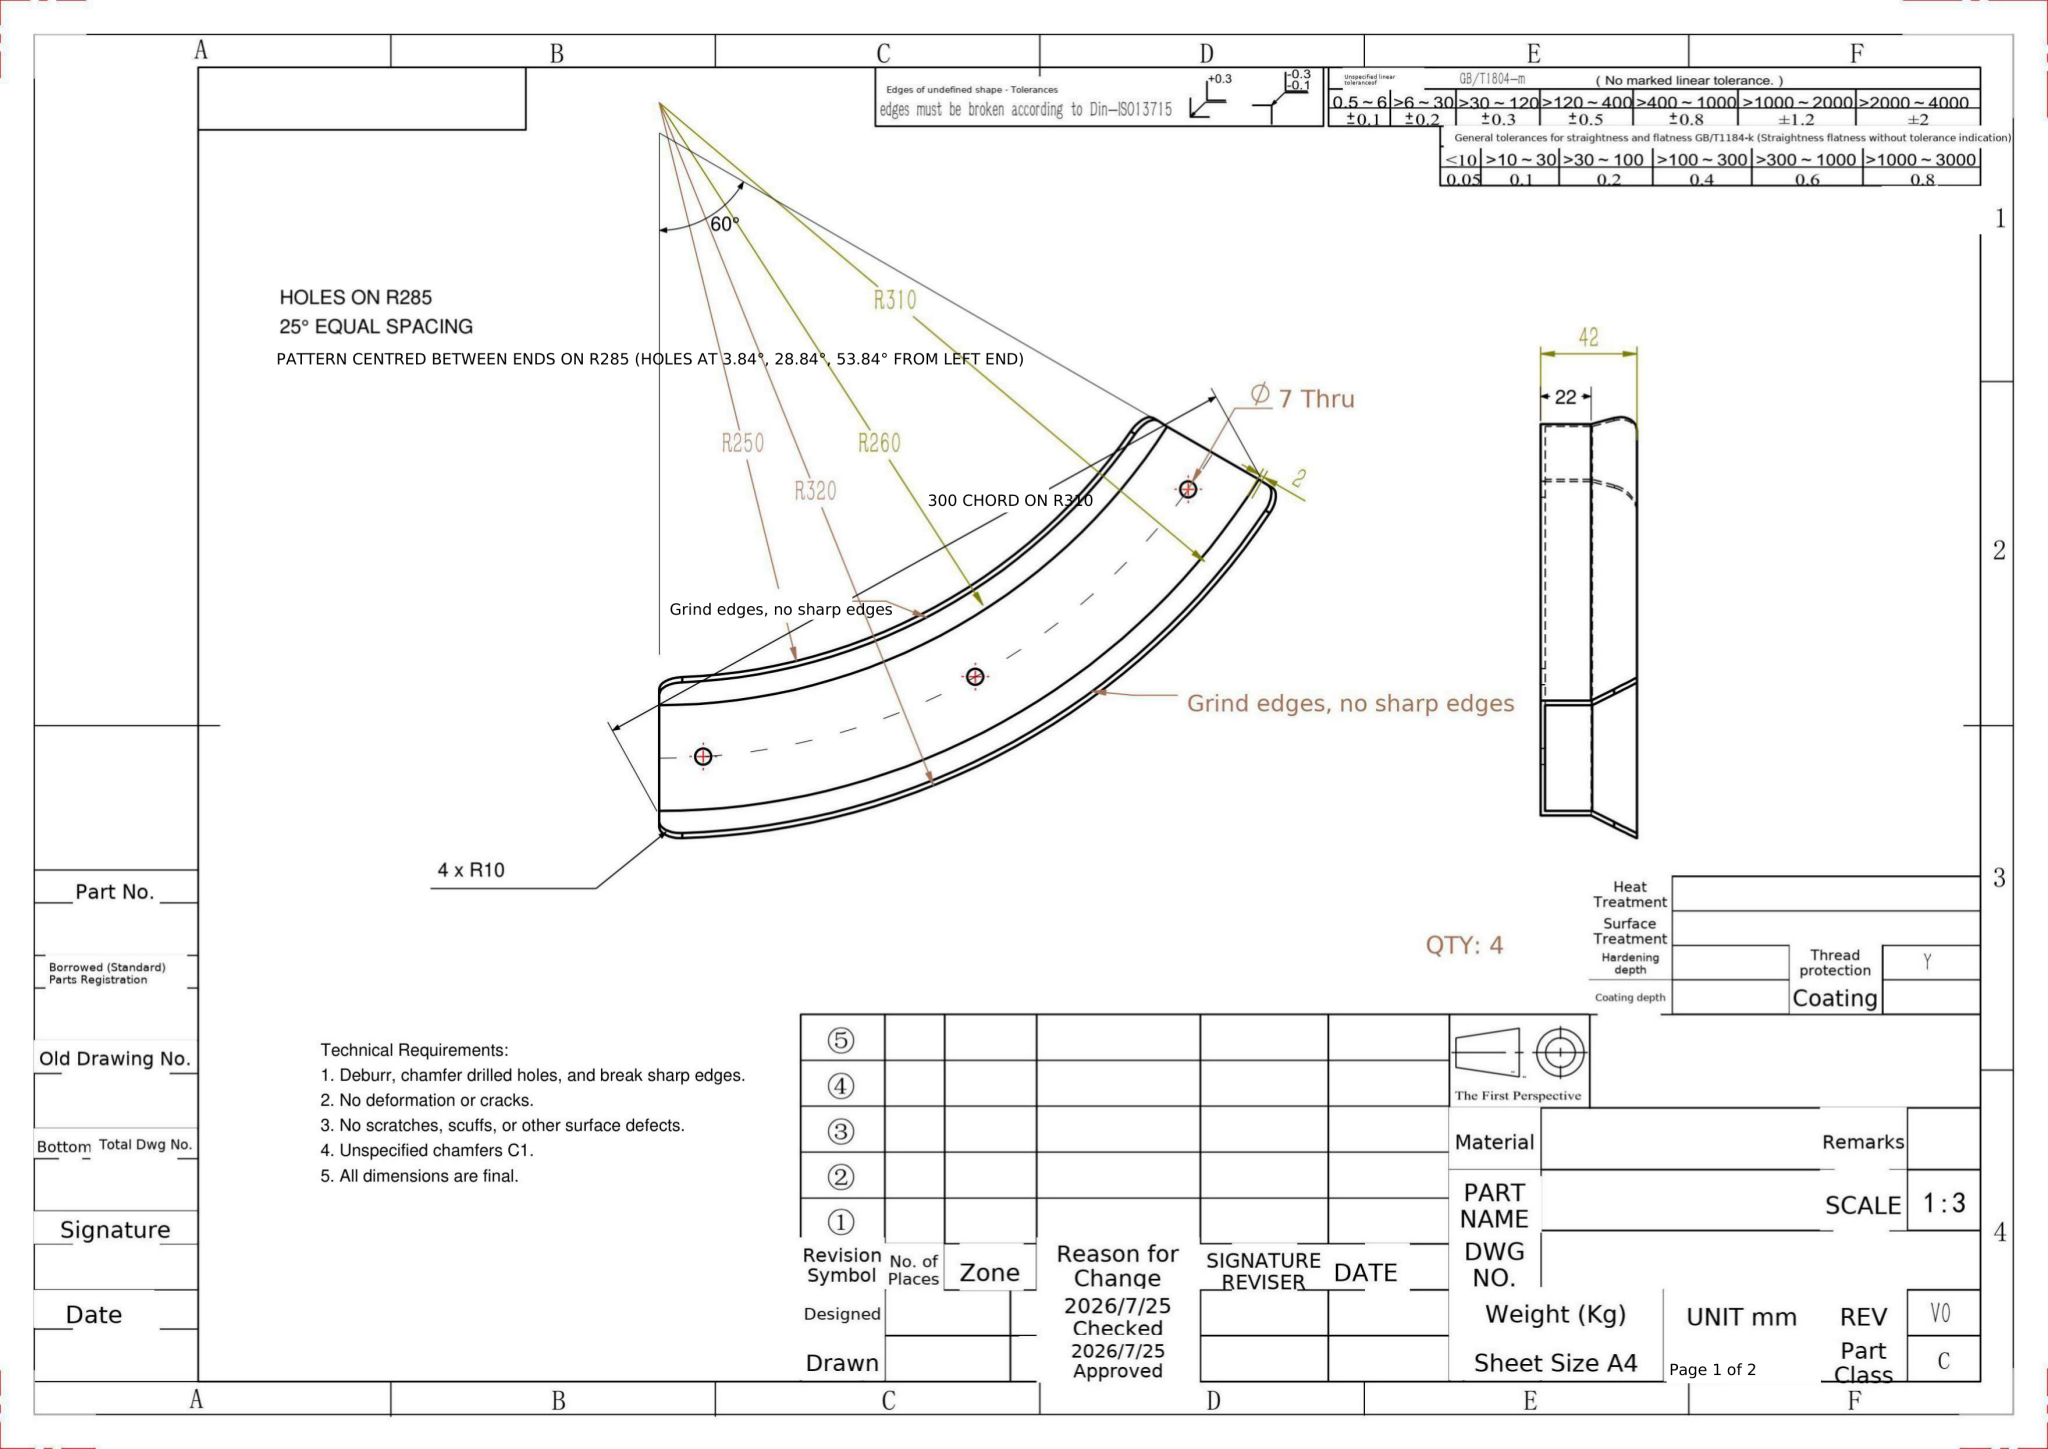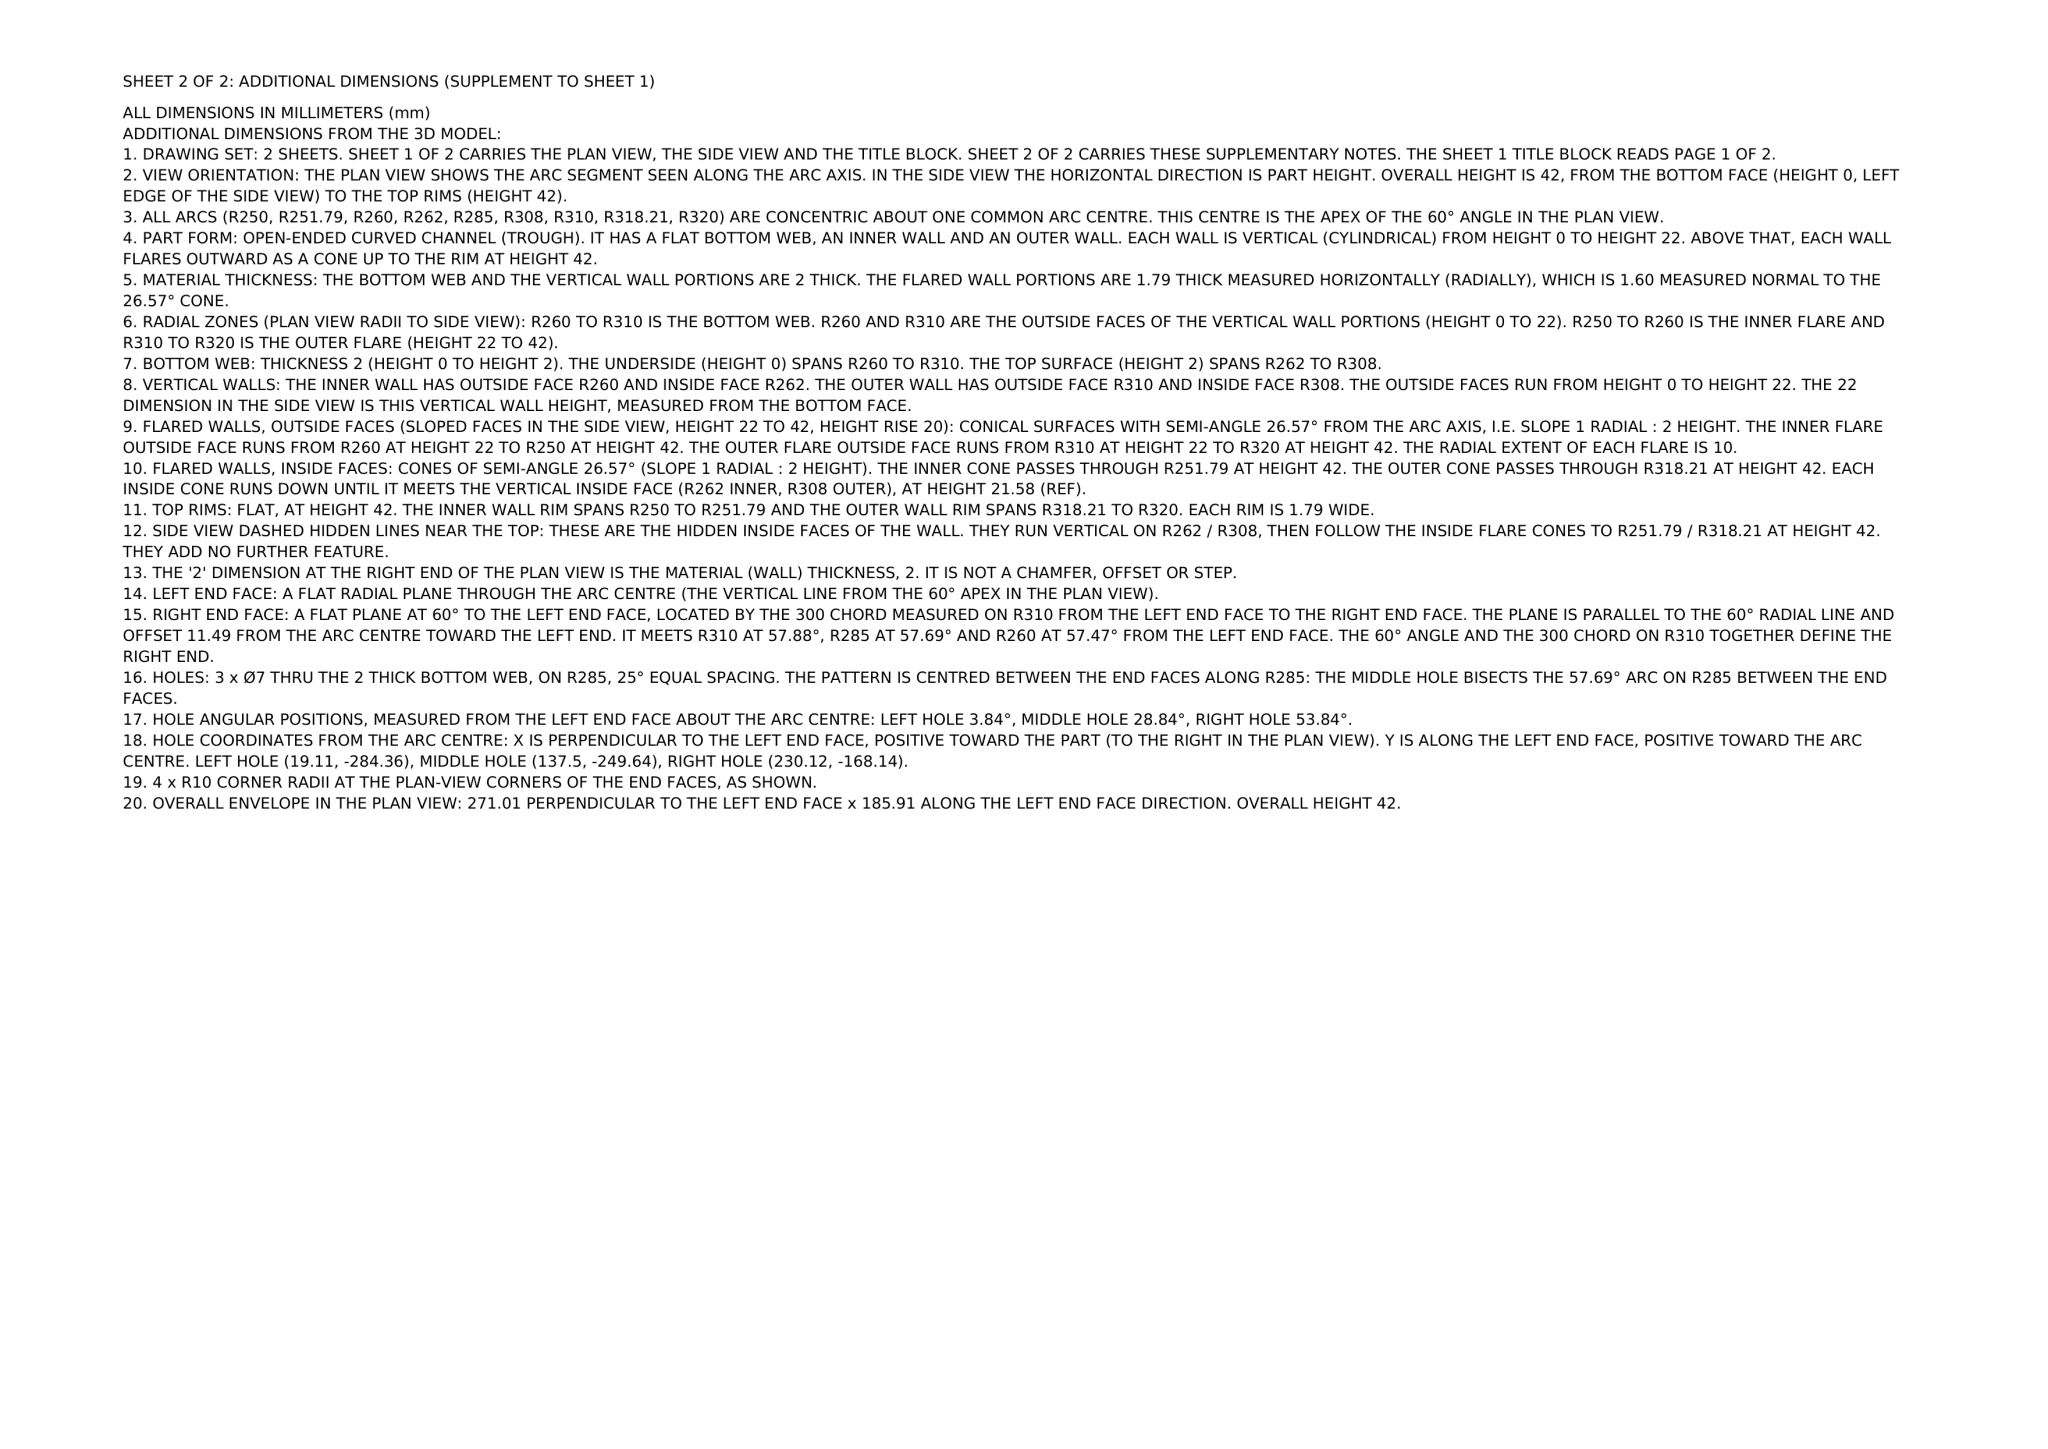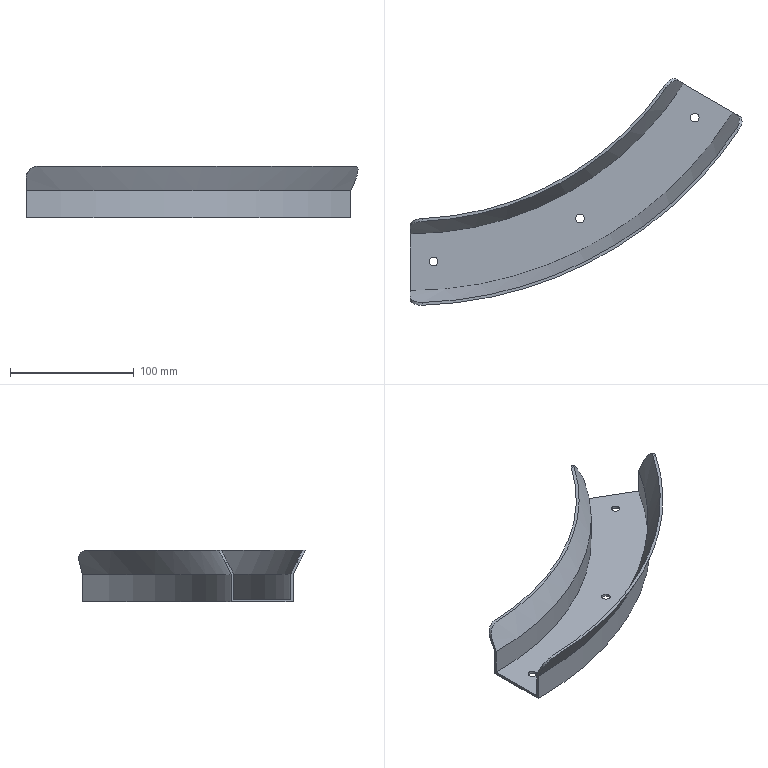Part | NX | mm | 1 solid | 26 faces | box 268.3 x 183.09 x 42 mm | volume 76866 mm3 | cylinder 12 | plane 6 | spline 4 | cone 4 | commonest cylinder face diameters 7 x6 20 x2 520 x1 620 x1 524 x1 616 x1